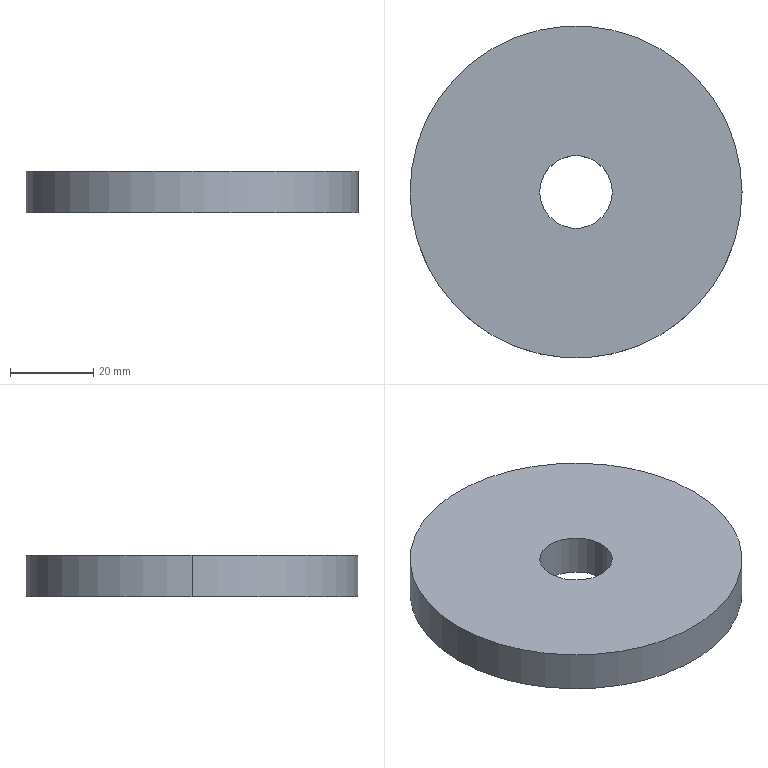Component | SolidWorks | YC1-250-02-28MotorSeatAssembly-1_YC1-250-02-25MotorShaftEndCover-1 | 1 solid | 6 faces | box 80 x 80 x 10 mm | volume 47860 mm3 | cylinder 4 | plane 2 | commonest cylinder face diameters 80 x2 17.5 x2 | material Plain Carbon Steel
STEP:
#1=COLOUR_RGB('',0.7922,0.8196,0.9333);
#2=FILL_AREA_STYLE_COLOUR('',#1);
#3=FILL_AREA_STYLE('',(#2));
#4=SURFACE_STYLE_FILL_AREA(#3);
#5=SURFACE_SIDE_STYLE('',(#4));
#6=SURFACE_STYLE_USAGE(.BOTH.,#5);
#7=PRESENTATION_STYLE_ASSIGNMENT((#6));
#8=CARTESIAN_POINT('',(1.575,151.181,-43.898));
#9=VERTEX_POINT('',#8);
#10=CARTESIAN_POINT('',(-1.575,151.181,-43.898));
#11=VERTEX_POINT('',#10);
#12=CARTESIAN_POINT('',(-0.,151.181,-43.898));
#13=DIRECTION('',(0.,0.,1.));
#14=DIRECTION('',(-1.,0.,0.));
#15=AXIS2_PLACEMENT_3D('',#12,#13,#14);
#16=CIRCLE('',#15,1.575);
#17=EDGE_CURVE('',#9,#11,#16,.T.);
#18=ORIENTED_EDGE('',*,*,#17,.F.);
#19=CARTESIAN_POINT('',(1.575,151.181,-44.291));
#20=VERTEX_POINT('',#19);
#21=CARTESIAN_POINT('',(1.575,151.181,-43.898));
#22=DIRECTION('',(0.,0.,-1.));
#23=VECTOR('',#22,39.37);
#24=LINE('',#21,#23);
#25=EDGE_CURVE('',#9,#20,#24,.T.);
#26=ORIENTED_EDGE('',*,*,#25,.T.);
#27=CARTESIAN_POINT('',(-1.575,151.181,-44.291));
#28=VERTEX_POINT('',#27);
#29=CARTESIAN_POINT('',(-0.,151.181,-44.291));
#30=DIRECTION('',(0.,0.,1.));
#31=DIRECTION('',(-1.,0.,0.));
#32=AXIS2_PLACEMENT_3D('',#29,#30,#31);
#33=CIRCLE('',#32,1.575);
#34=EDGE_CURVE('',#20,#28,#33,.T.);
#35=ORIENTED_EDGE('',*,*,#34,.T.);
#36=CARTESIAN_POINT('',(-1.575,151.181,-43.898));
#37=DIRECTION('',(0.,0.,-1.));
#38=VECTOR('',#37,39.37);
#39=LINE('',#36,#38);
#40=EDGE_CURVE('',#11,#28,#39,.T.);
#41=ORIENTED_EDGE('',*,*,#40,.F.);
#42=EDGE_LOOP('',(#18,#26,#35,#41));
#43=FACE_OUTER_BOUND('',#42,.T.);
#44=CARTESIAN_POINT('',(-0.,151.181,-43.898));
#45=DIRECTION('',(0.,0.,-1.));
#46=DIRECTION('',(-1.,0.,0.));
#47=AXIS2_PLACEMENT_3D('',#44,#45,#46);
#48=CYLINDRICAL_SURFACE('',#47,1.575);
#49=ADVANCED_FACE('',(#43),#48,.T.);
#50=CARTESIAN_POINT('',(-0.3445,151.181,-44.291));
#51=VERTEX_POINT('',#50);
#52=CARTESIAN_POINT('',(0.3445,151.181,-44.291));
#53=VERTEX_POINT('',#52);
#54=CARTESIAN_POINT('',(-0.,151.181,-44.291));
#55=DIRECTION('',(0.,0.,1.));
#56=DIRECTION('',(1.,0.,0.));
#57=AXIS2_PLACEMENT_3D('',#54,#55,#56);
#58=CIRCLE('',#57,0.3445);
#59=EDGE_CURVE('',#51,#53,#58,.T.);
#60=ORIENTED_EDGE('',*,*,#59,.F.);
#61=CARTESIAN_POINT('',(-0.3445,151.181,-43.898));
#62=VERTEX_POINT('',#61);
#63=CARTESIAN_POINT('',(-0.3445,151.181,-43.898));
#64=DIRECTION('',(0.,0.,1.));
#65=VECTOR('',#64,39.37);
#66=LINE('',#63,#65);
#67=EDGE_CURVE('',#51,#62,#66,.T.);
#68=ORIENTED_EDGE('',*,*,#67,.T.);
#69=CARTESIAN_POINT('',(0.3445,151.181,-43.898));
#70=VERTEX_POINT('',#69);
#71=CARTESIAN_POINT('',(-0.,151.181,-43.898));
#72=DIRECTION('',(0.,0.,-1.));
#73=DIRECTION('',(1.,0.,0.));
#74=AXIS2_PLACEMENT_3D('',#71,#72,#73);
#75=CIRCLE('',#74,0.3445);
#76=EDGE_CURVE('',#70,#62,#75,.T.);
#77=ORIENTED_EDGE('',*,*,#76,.F.);
#78=CARTESIAN_POINT('',(0.3445,151.181,-43.898));
#79=DIRECTION('',(0.,0.,1.));
#80=VECTOR('',#79,39.37);
#81=LINE('',#78,#80);
#82=EDGE_CURVE('',#53,#70,#81,.T.);
#83=ORIENTED_EDGE('',*,*,#82,.F.);
#84=EDGE_LOOP('',(#60,#68,#77,#83));
#85=FACE_OUTER_BOUND('',#84,.T.);
#86=CARTESIAN_POINT('',(-0.,151.181,-43.898));
#87=DIRECTION('',(0.,0.,1.));
#88=DIRECTION('',(1.,0.,0.));
#89=AXIS2_PLACEMENT_3D('',#86,#87,#88);
#90=CYLINDRICAL_SURFACE('',#89,0.3445);
#91=ADVANCED_FACE('',(#85),#90,.F.);
#92=CARTESIAN_POINT('',(-0.,151.181,-43.898));
#93=DIRECTION('',(0.,0.,1.));
#94=DIRECTION('',(-1.,0.,0.));
#95=AXIS2_PLACEMENT_3D('',#92,#93,#94);
#96=CIRCLE('',#95,1.575);
#97=EDGE_CURVE('',#11,#9,#96,.T.);
#98=ORIENTED_EDGE('',*,*,#97,.T.);
#99=ORIENTED_EDGE('',*,*,#17,.T.);
#100=EDGE_LOOP('',(#98,#99));
#101=FACE_OUTER_BOUND('',#100,.T.);
#102=ORIENTED_EDGE('',*,*,#76,.T.);
#103=CARTESIAN_POINT('',(-0.,151.181,-43.898));
#104=DIRECTION('',(0.,0.,-1.));
#105=DIRECTION('',(1.,0.,0.));
#106=AXIS2_PLACEMENT_3D('',#103,#104,#105);
#107=CIRCLE('',#106,0.3445);
#108=EDGE_CURVE('',#62,#70,#107,.T.);
#109=ORIENTED_EDGE('',*,*,#108,.T.);
#110=EDGE_LOOP('',(#102,#109));
#111=FACE_BOUND('',#110,.T.);
#112=CARTESIAN_POINT('',(-0.,151.181,-43.898));
#113=DIRECTION('',(0.,0.,1.));
#114=DIRECTION('',(1.,0.,0.));
#115=AXIS2_PLACEMENT_3D('',#112,#113,#114);
#116=PLANE('',#115);
#117=ADVANCED_FACE('',(#101,#111),#116,.T.);
#118=ORIENTED_EDGE('',*,*,#25,.F.);
#119=ORIENTED_EDGE('',*,*,#97,.F.);
#120=ORIENTED_EDGE('',*,*,#40,.T.);
#121=CARTESIAN_POINT('',(-0.,151.181,-44.291));
#122=DIRECTION('',(0.,0.,1.));
#123=DIRECTION('',(-1.,0.,0.));
#124=AXIS2_PLACEMENT_3D('',#121,#122,#123);
#125=CIRCLE('',#124,1.575);
#126=EDGE_CURVE('',#28,#20,#125,.T.);
#127=ORIENTED_EDGE('',*,*,#126,.T.);
#128=EDGE_LOOP('',(#118,#119,#120,#127));
#129=FACE_OUTER_BOUND('',#128,.T.);
#130=CARTESIAN_POINT('',(-0.,151.181,-43.898));
#131=DIRECTION('',(0.,0.,-1.));
#132=DIRECTION('',(-1.,0.,0.));
#133=AXIS2_PLACEMENT_3D('',#130,#131,#132);
#134=CYLINDRICAL_SURFACE('',#133,1.575);
#135=ADVANCED_FACE('',(#129),#134,.T.);
#136=ORIENTED_EDGE('',*,*,#67,.F.);
#137=CARTESIAN_POINT('',(-0.,151.181,-44.291));
#138=DIRECTION('',(0.,0.,1.));
#139=DIRECTION('',(1.,0.,0.));
#140=AXIS2_PLACEMENT_3D('',#137,#138,#139);
#141=CIRCLE('',#140,0.3445);
#142=EDGE_CURVE('',#53,#51,#141,.T.);
#143=ORIENTED_EDGE('',*,*,#142,.F.);
#144=ORIENTED_EDGE('',*,*,#82,.T.);
#145=ORIENTED_EDGE('',*,*,#108,.F.);
#146=EDGE_LOOP('',(#136,#143,#144,#145));
#147=FACE_OUTER_BOUND('',#146,.T.);
#148=CARTESIAN_POINT('',(-0.,151.181,-43.898));
#149=DIRECTION('',(0.,0.,1.));
#150=DIRECTION('',(1.,0.,0.));
#151=AXIS2_PLACEMENT_3D('',#148,#149,#150);
#152=CYLINDRICAL_SURFACE('',#151,0.3445);
#153=ADVANCED_FACE('',(#147),#152,.F.);
#154=ORIENTED_EDGE('',*,*,#126,.F.);
#155=ORIENTED_EDGE('',*,*,#34,.F.);
#156=EDGE_LOOP('',(#154,#155));
#157=FACE_OUTER_BOUND('',#156,.T.);
#158=ORIENTED_EDGE('',*,*,#142,.T.);
#159=ORIENTED_EDGE('',*,*,#59,.T.);
#160=EDGE_LOOP('',(#158,#159));
#161=FACE_BOUND('',#160,.T.);
#162=CARTESIAN_POINT('',(-0.,151.181,-44.291));
#163=DIRECTION('',(0.,0.,1.));
#164=DIRECTION('',(1.,0.,0.));
#165=AXIS2_PLACEMENT_3D('',#162,#163,#164);
#166=PLANE('',#165);
#167=ADVANCED_FACE('',(#157,#161),#166,.F.);
#168=CLOSED_SHELL('',(#49,#91,#117,#135,#153,#167));
#169=MANIFOLD_SOLID_BREP('',#168);
#170=STYLED_ITEM('',(#7),#169);
#171=(LENGTH_UNIT()NAMED_UNIT(*)SI_UNIT($,.METRE.));
#172=LENGTH_MEASURE_WITH_UNIT(LENGTH_MEASURE(0.0254),#171);
#173=DIMENSIONAL_EXPONENTS(1.,0.,0.,0.,0.,0.,0.);
#174=(CONVERSION_BASED_UNIT('',#172)LENGTH_UNIT()NAMED_UNIT(#173));
#175=UNCERTAINTY_MEASURE_WITH_UNIT(LENGTH_MEASURE(0.00001),#174,'','');
#176=(NAMED_UNIT(*)PLANE_ANGLE_UNIT()SI_UNIT($,.RADIAN.));
#177=(NAMED_UNIT(*)SI_UNIT($,.STERADIAN.)SOLID_ANGLE_UNIT());
#178=(GEOMETRIC_REPRESENTATION_CONTEXT(3)GLOBAL_UNCERTAINTY_ASSIGNED_CONTEXT((#175))GLOBAL_UNIT_ASSIGNED_CONTEXT((#174,#176,#177))REPRESENTATION_CONTEXT('',''));
#179=MECHANICAL_DESIGN_GEOMETRIC_PRESENTATION_REPRESENTATION('',(#170),#178);
#180=CARTESIAN_POINT('',(0.,0.,0.));
#181=DIRECTION('',(0.,0.,1.));
#182=DIRECTION('',(1.,0.,0.));
#183=AXIS2_PLACEMENT_3D('',#180,#181,#182);
#184=(LENGTH_UNIT()NAMED_UNIT(*)SI_UNIT($,.METRE.));
#185=LENGTH_MEASURE_WITH_UNIT(LENGTH_MEASURE(0.0254),#184);
#186=DIMENSIONAL_EXPONENTS(1.,0.,0.,0.,0.,0.,0.);
#187=(CONVERSION_BASED_UNIT('',#185)LENGTH_UNIT()NAMED_UNIT(#186));
#188=UNCERTAINTY_MEASURE_WITH_UNIT(LENGTH_MEASURE(0.00001),#187,'','');
#189=(NAMED_UNIT(*)PLANE_ANGLE_UNIT()SI_UNIT($,.RADIAN.));
#190=(NAMED_UNIT(*)SI_UNIT($,.STERADIAN.)SOLID_ANGLE_UNIT());
#191=(GEOMETRIC_REPRESENTATION_CONTEXT(3)GLOBAL_UNCERTAINTY_ASSIGNED_CONTEXT((#188))GLOBAL_UNIT_ASSIGNED_CONTEXT((#187,#189,#190))REPRESENTATION_CONTEXT('',''));
#192=ADVANCED_BREP_SHAPE_REPRESENTATION('',(#169,#183),#191);
#193=PRESENTATION_LAYER_ASSIGNMENT('','',(#170));